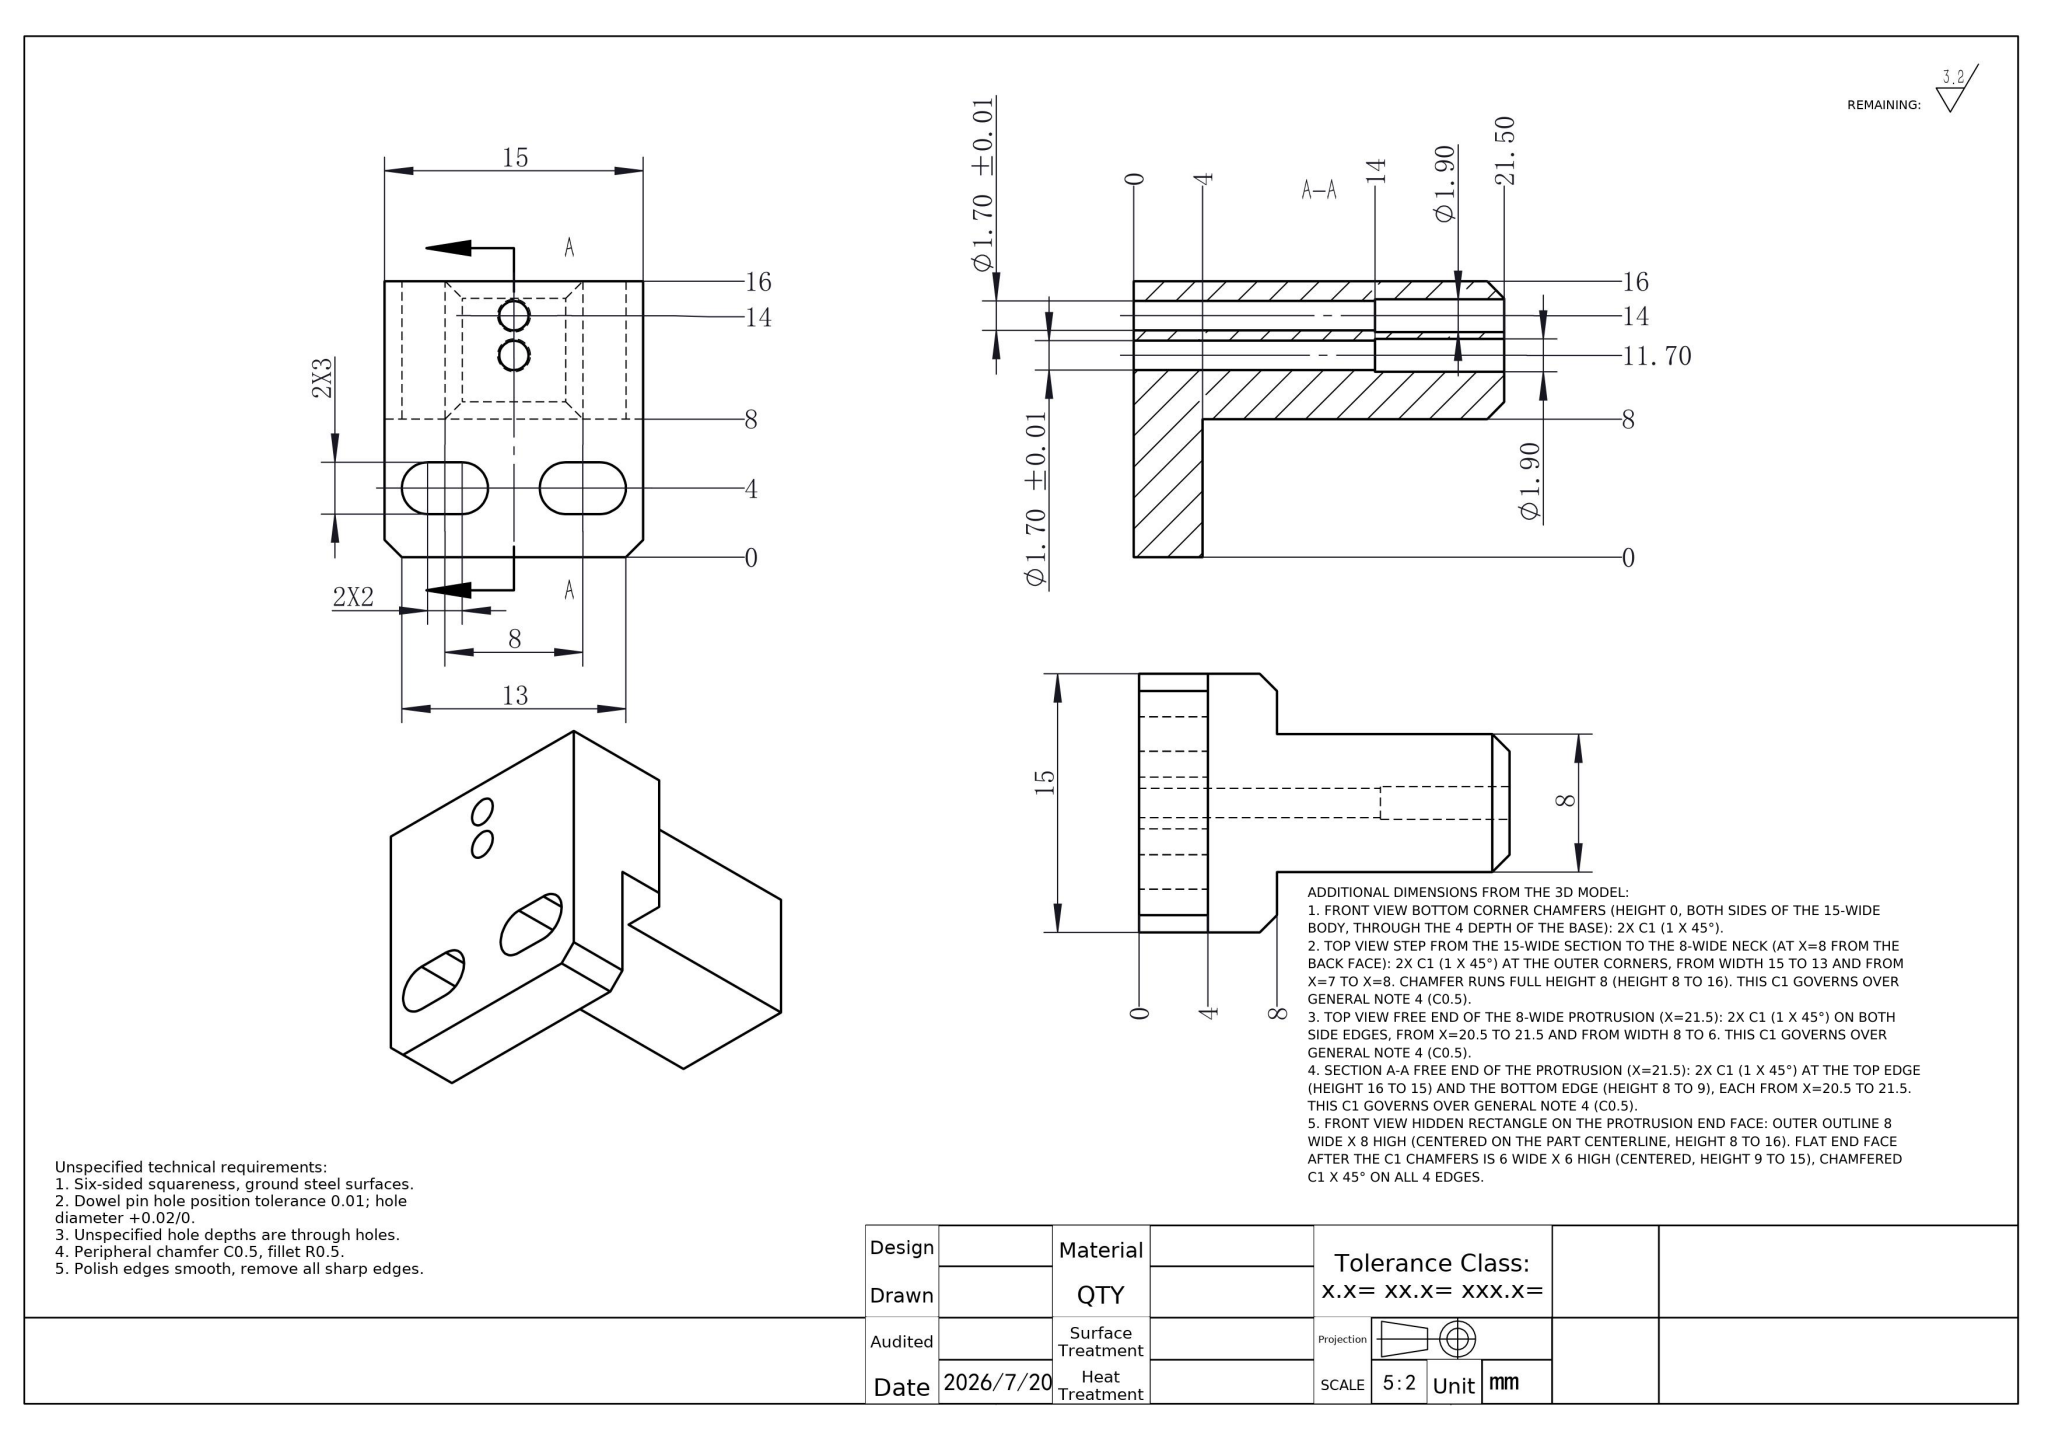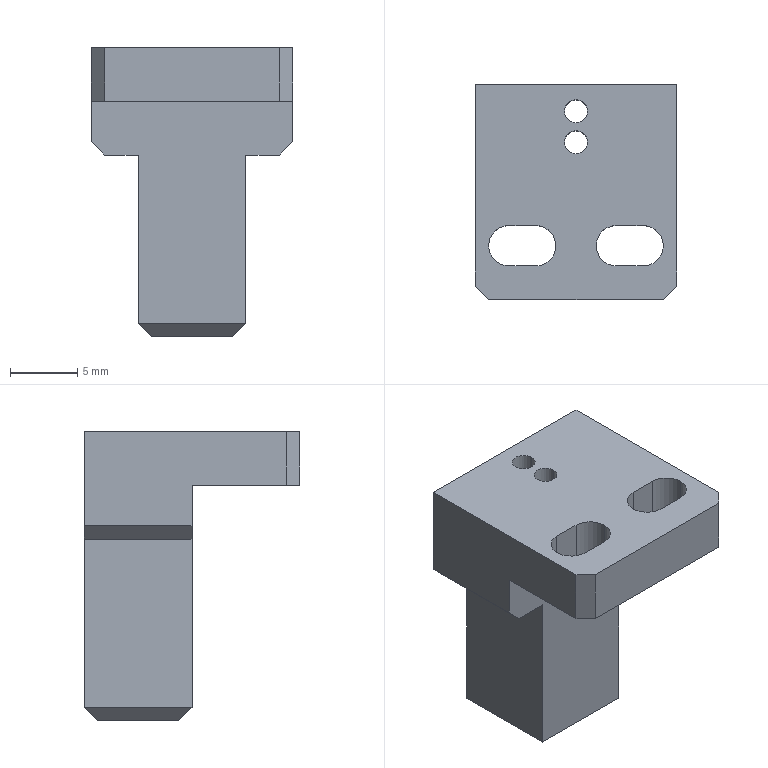Part | NX | mm | 1 solid | 40 faces | box 15 x 16 x 21.5 mm | volume 2067 mm3 | plane 26 | cylinder 14 | commonest cylinder face diameters 3 x6 1.9 x4 1.7 x4